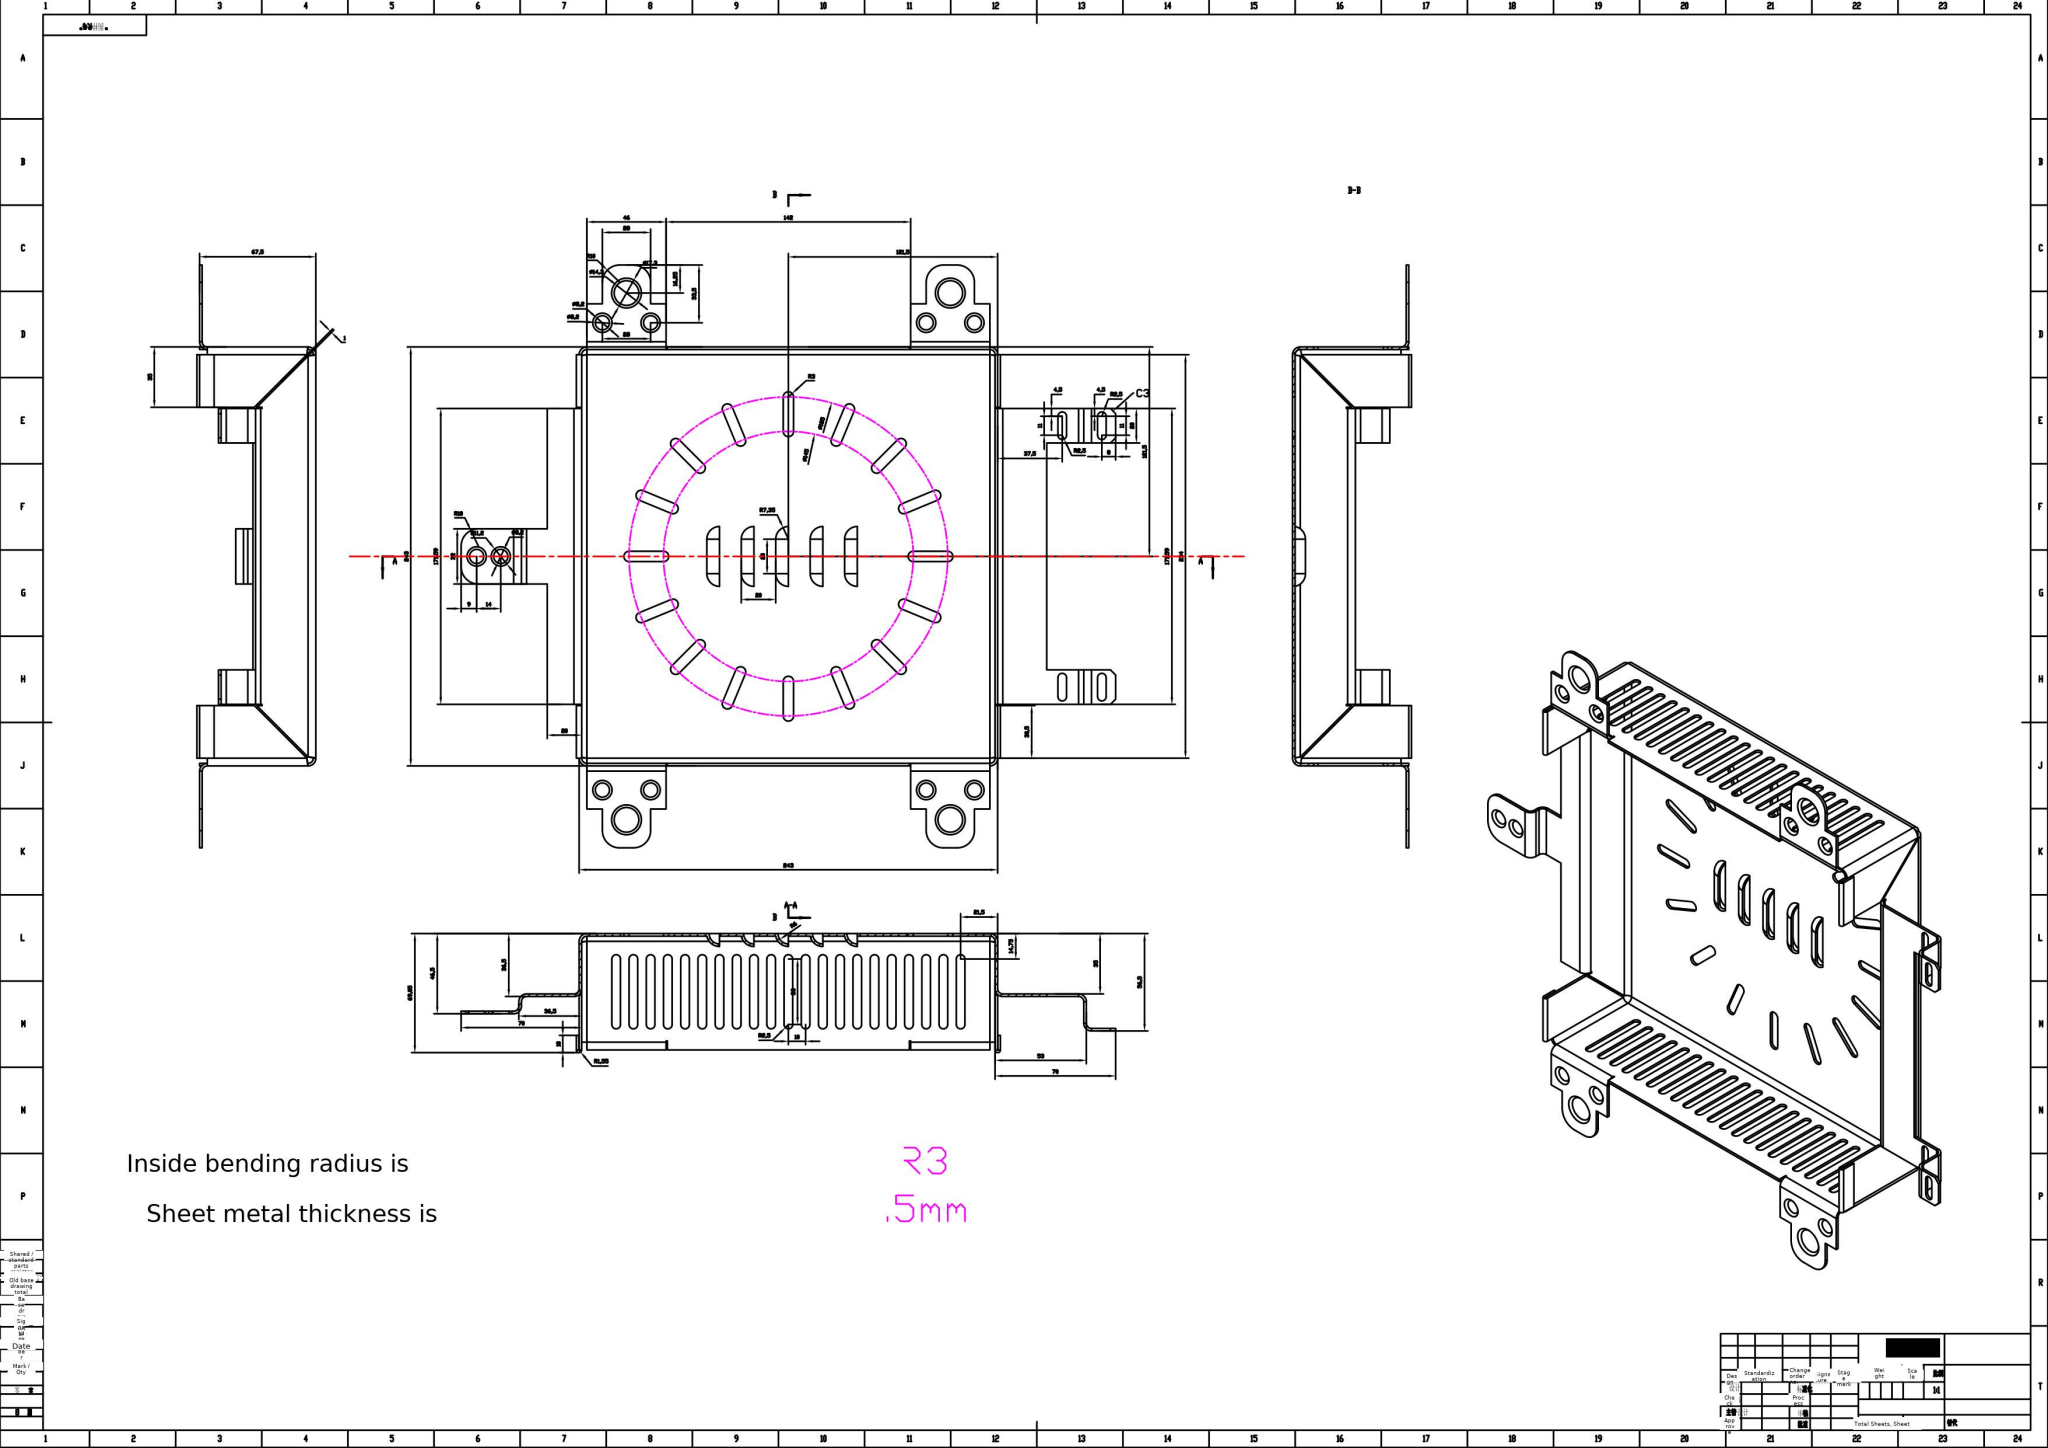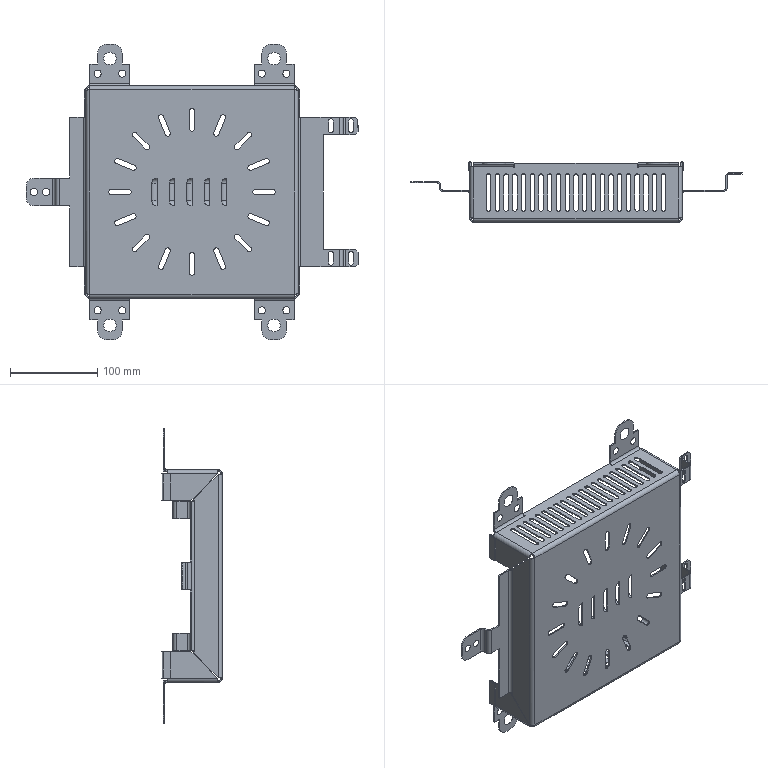Part | SolidWorks | 1 solid | 598 faces | box 380 x 69.05 x 338 mm | volume 175186 mm3 | plane 336 | cylinder 206 | cone 28 | sphere 20 | spline 8 | commonest cylinder face diameters 5 x92 6 x66 9 x20 20 x10 12 x5 15 x5 3.1 x4 0.1 x4